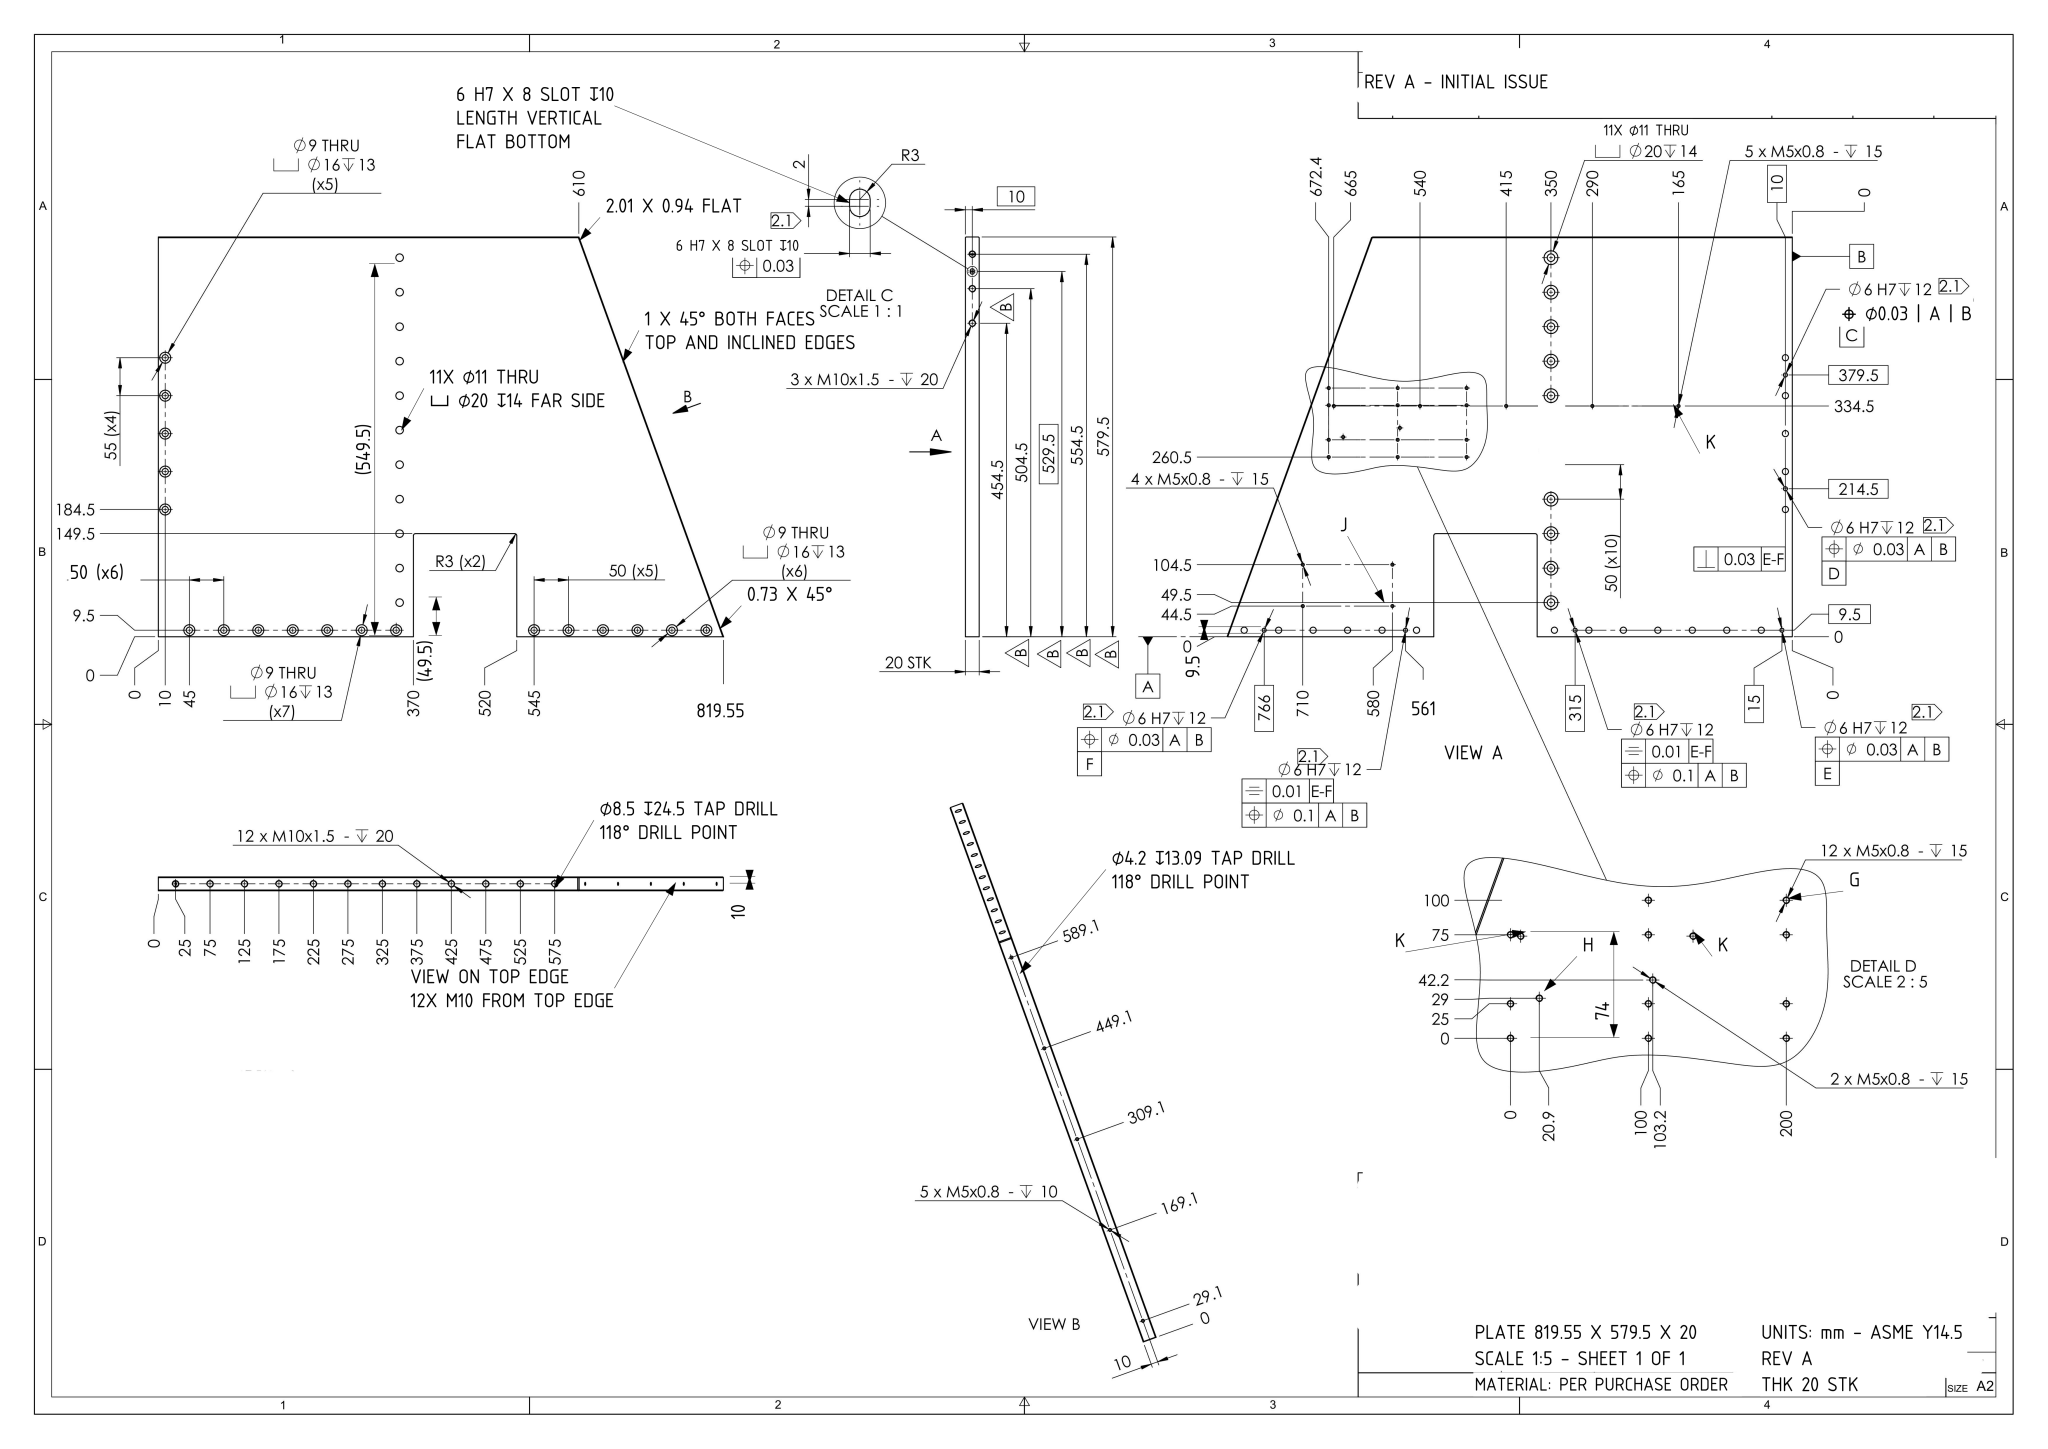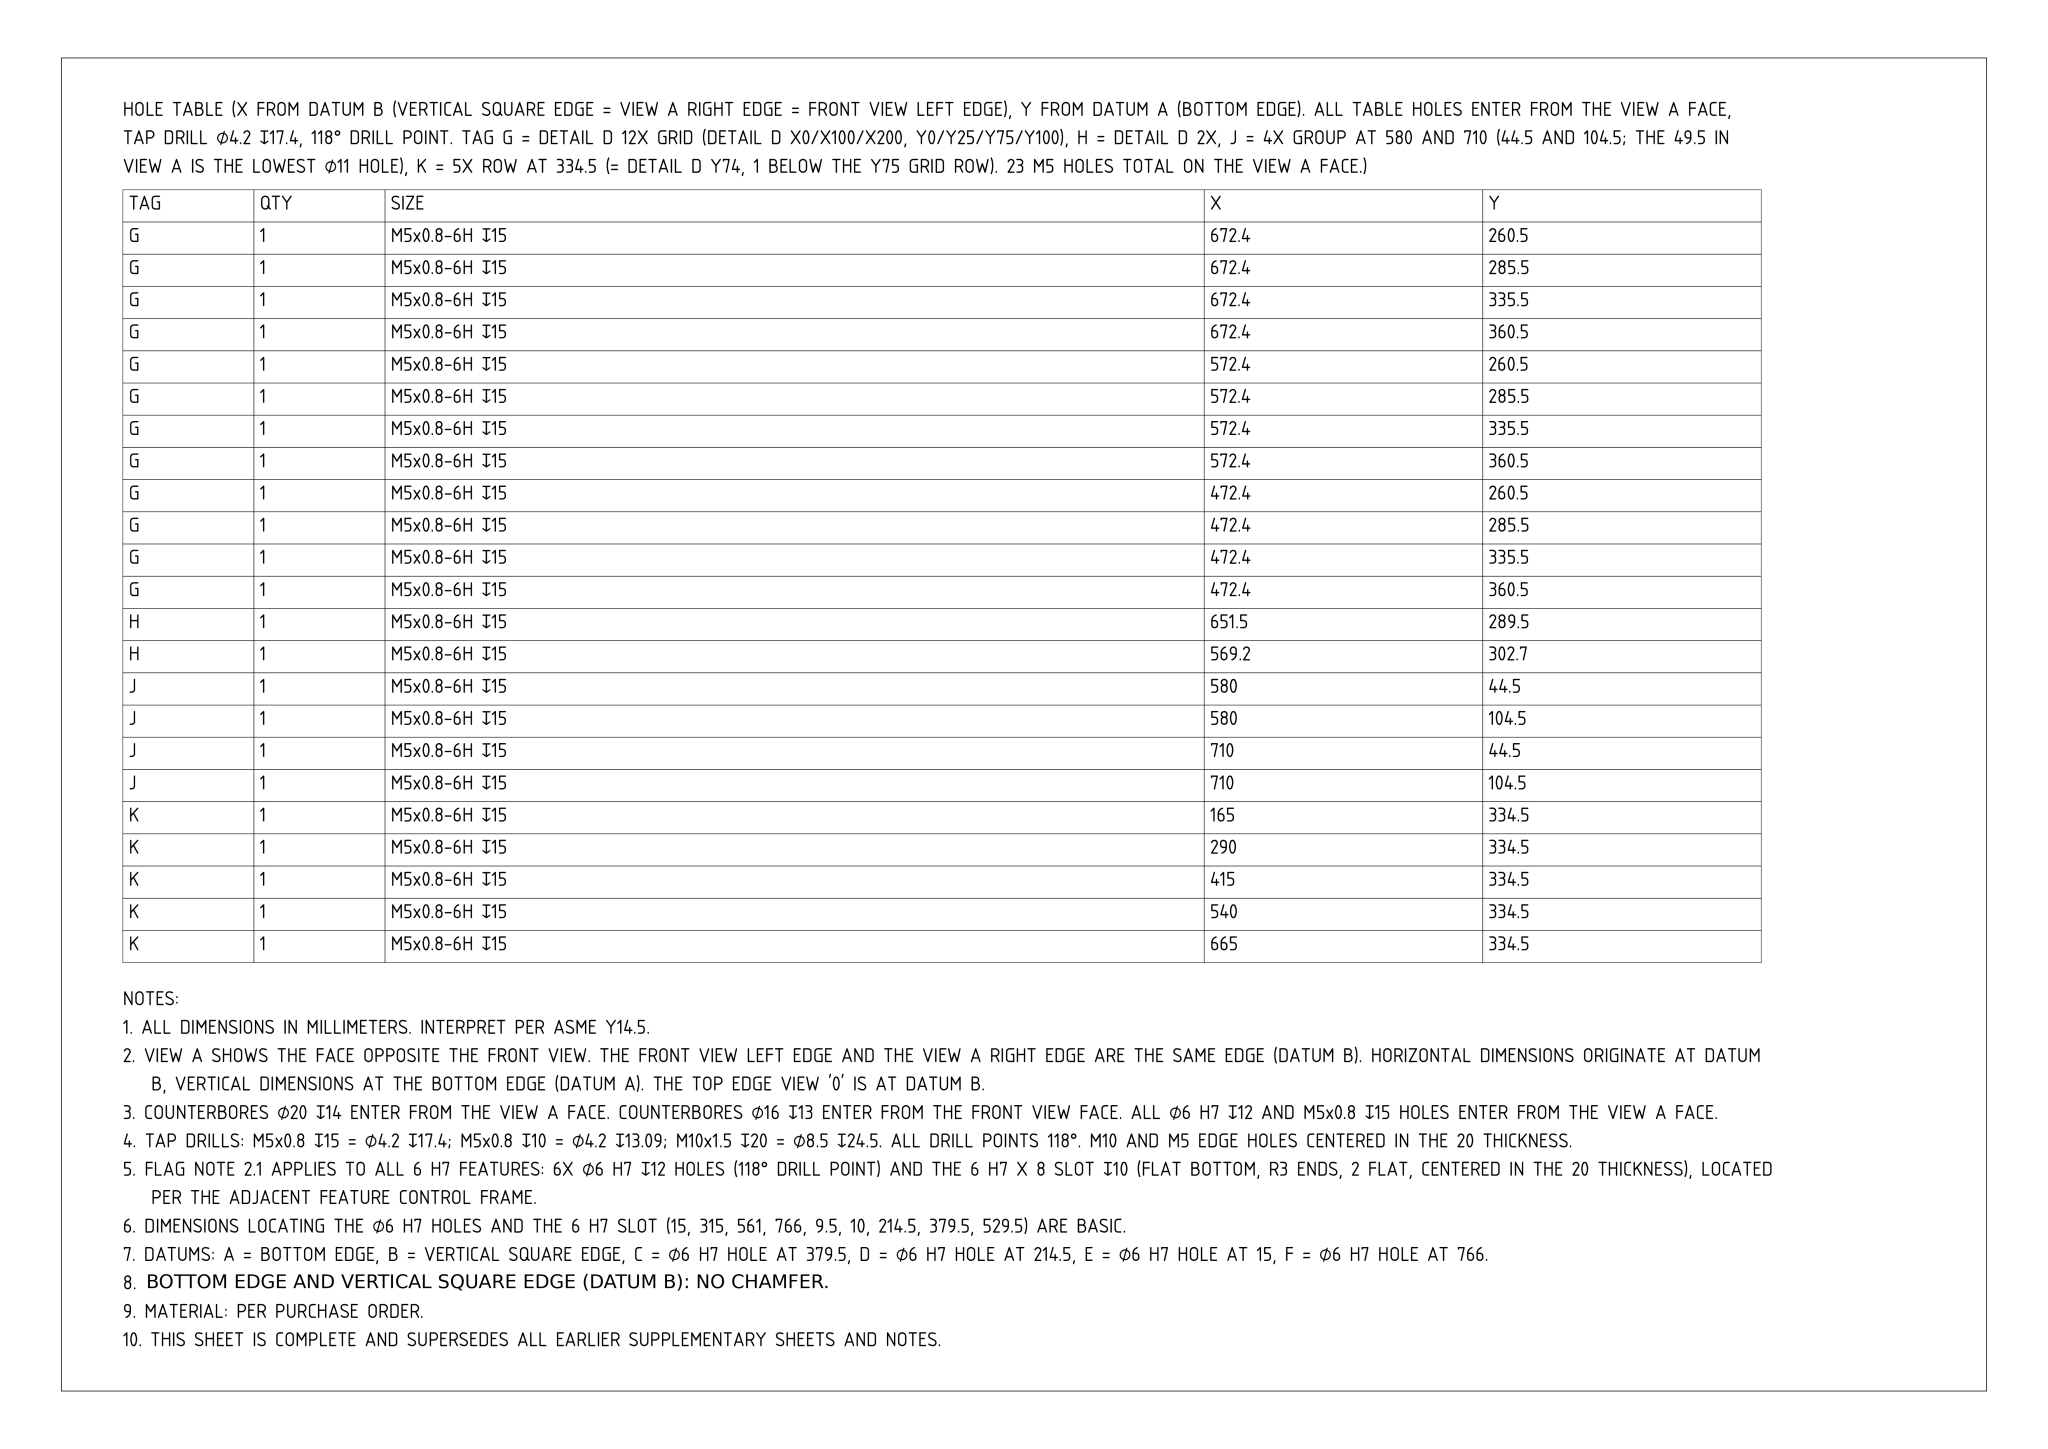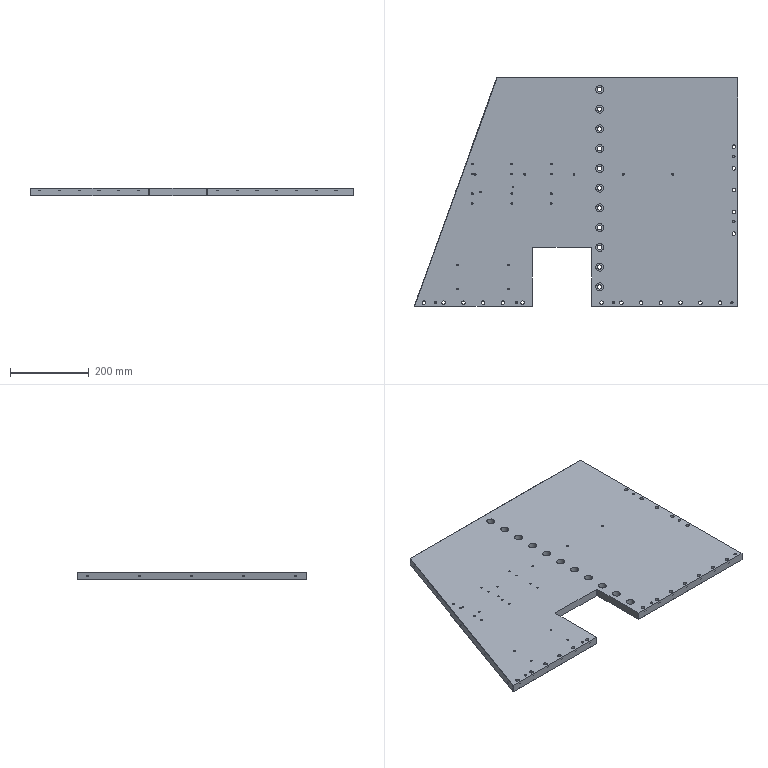Part | NX | mm | 1 solid | 368 faces | box 819.55 x 579.5 x 20 mm | volume 7695859 mm3 | cylinder 218 | cone 100 | plane 50 | commonest cylinder face diameters 4.2 x56 9 x36 16 x36 8.5 x30 20 x22 11 x22 6 x16